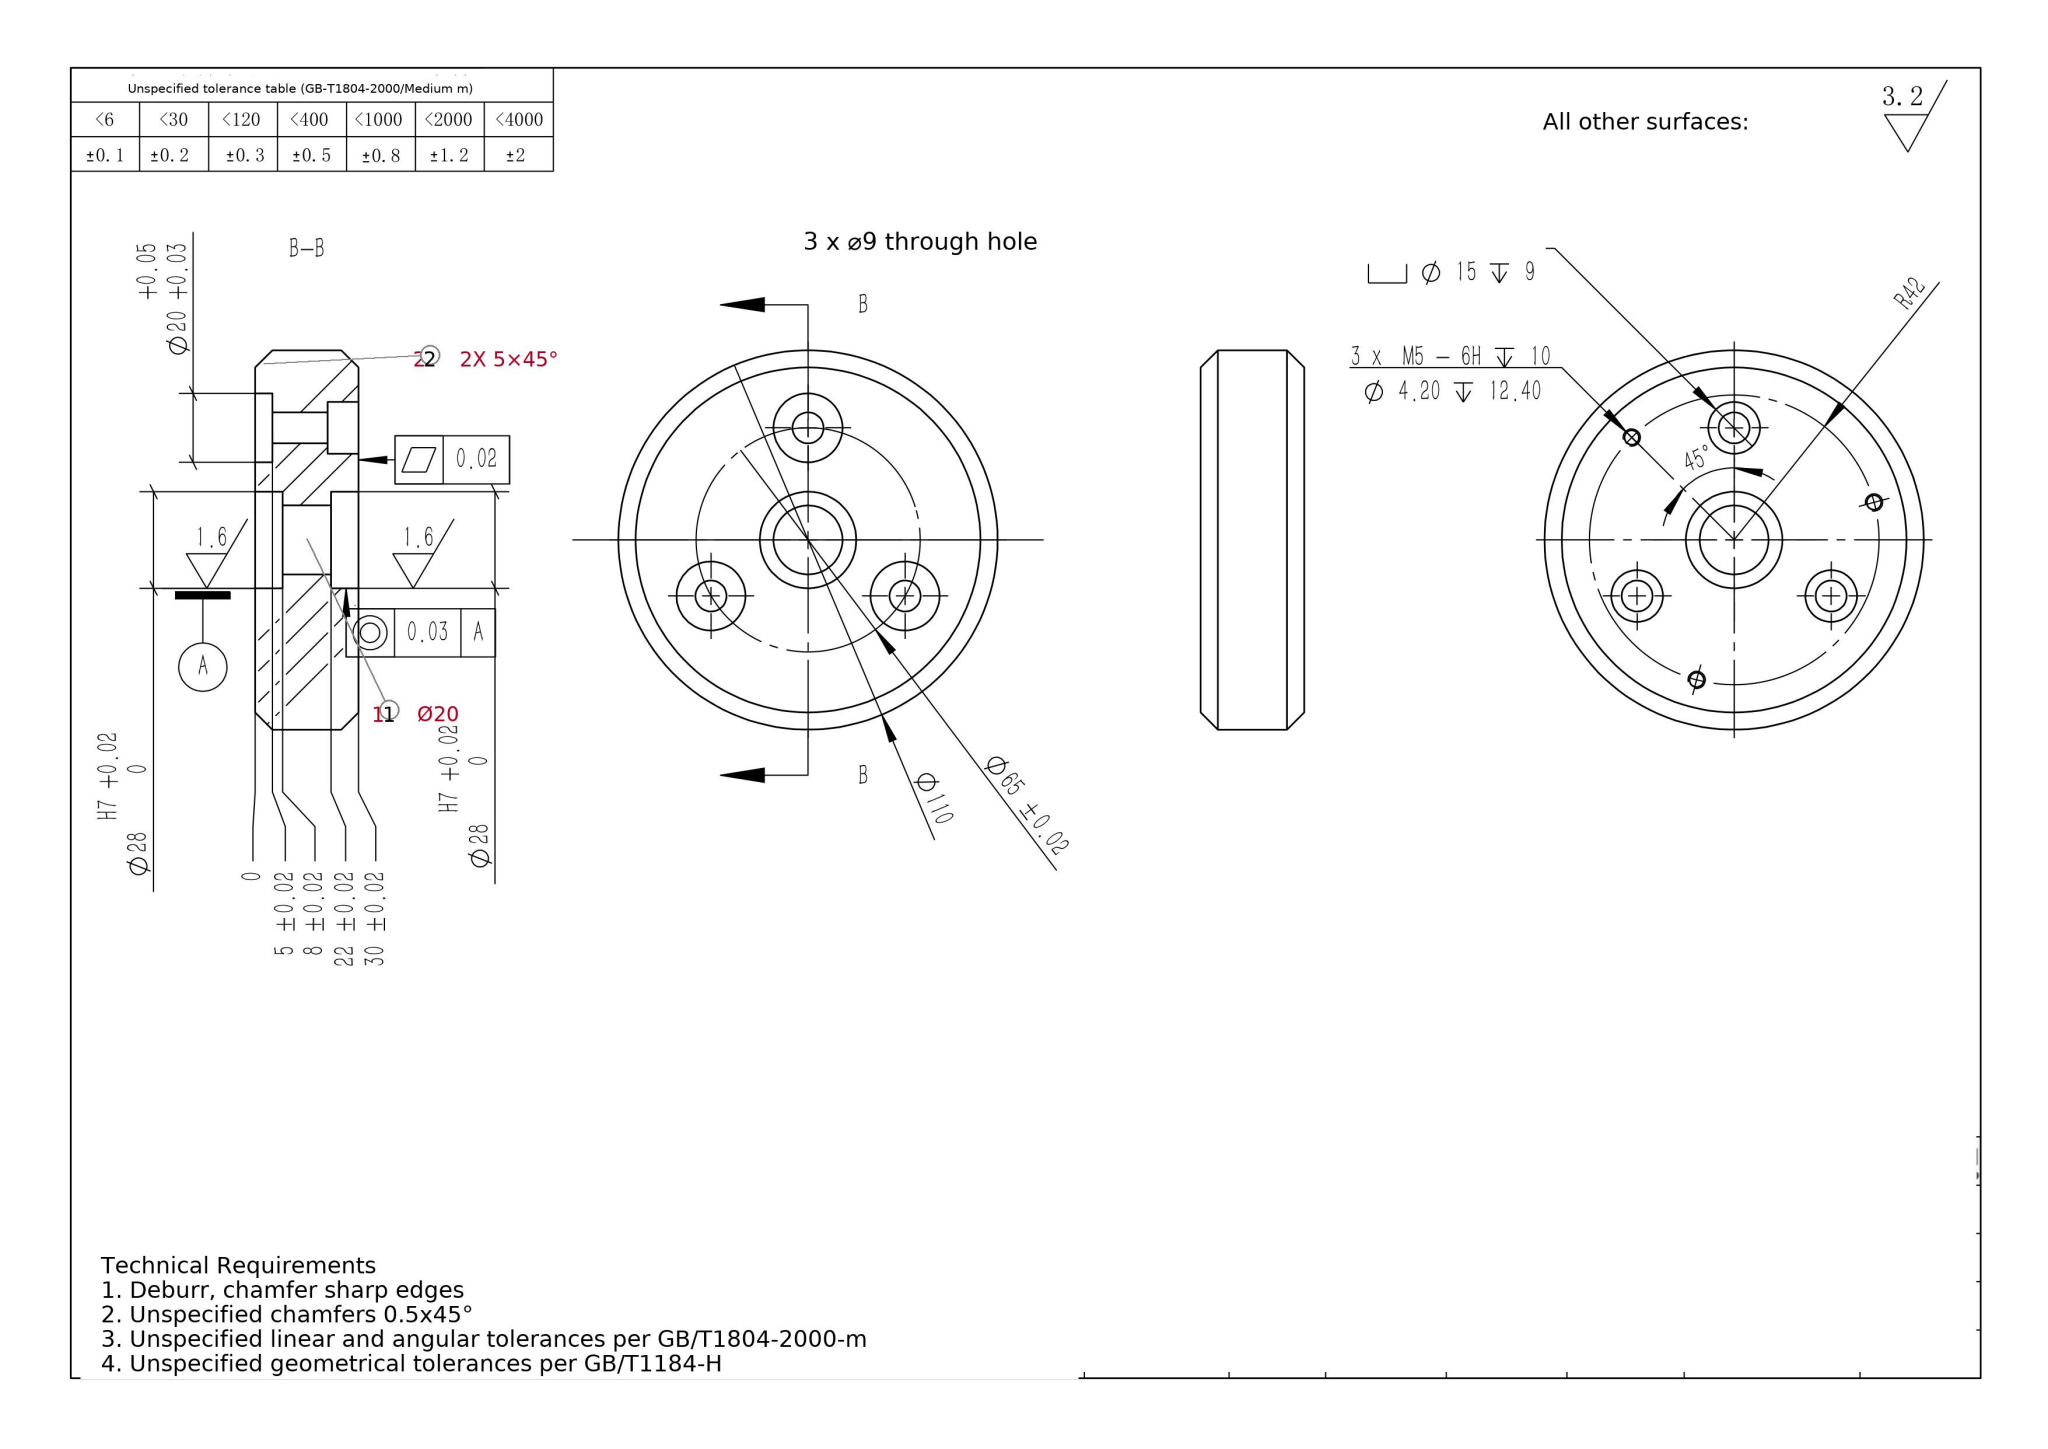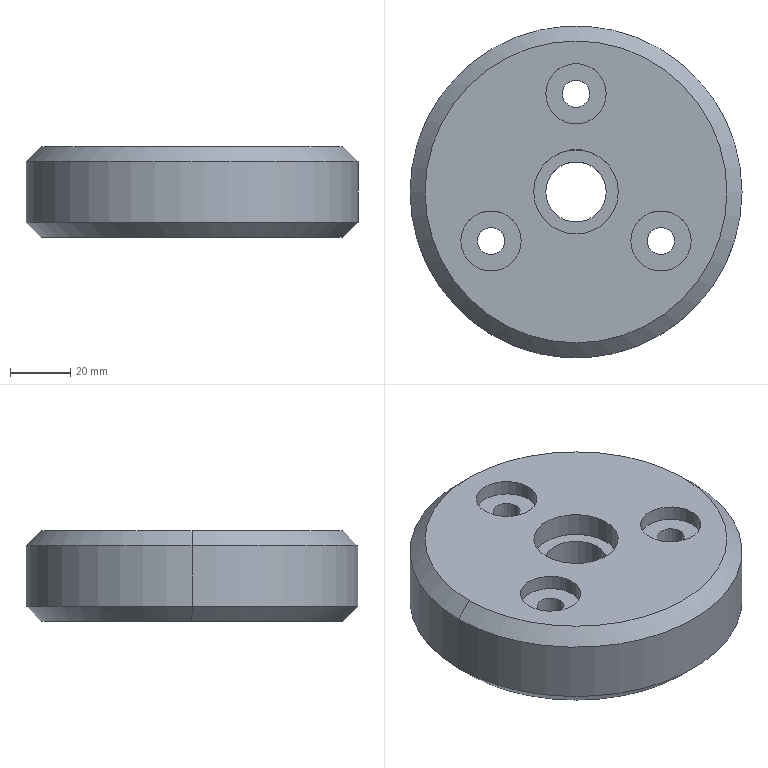Part | SolidWorks | mm | 1 solid | 52 faces | box 110 x 110 x 30 mm | volume 249402 mm3 | cylinder 32 | cone 10 | plane 10 | commonest cylinder face diameters 20 x8 4.2 x6 15 x6 9 x6 28 x4 110 x2
build123d program:
from build123d import *

# Parameters (mm, degrees)
SKETCH1_R                                         = 55
BOSS_EXTRUDE1_DEPTH                               = 30
SKETCH2_R                                         = 14
CUT_EXTRUDE1_DEPTH                                = 8
SKETCH3_R                                         = 10
CUT_EXTRUDE2_DEPTH                                = 81.833
CUT_EXTRUDE3_START                                = -8
SKETCH4_R                                         = 14
CUT_EXTRUDE3_DEPTH                                = 8
SKETCH5_R                                         = 10
CUT_EXTRUDE4_DEPTH                                = 5
HOLE_SIZE_ACCORDING_TO_HEXAGON_SOCKET_D           = 9
HOLE_SIZE_ACCORDING_TO_HEXAGON_SOCKET_CBORE_D     = 15
HOLE_SIZE_ACCORDING_TO_HEXAGON_SOCKET_CBORE_DEPTH = 9
CHAMFER1_SIZE                                     = 5
M5_TAPPED_HOLE1_D                                 = 4.2
M5_TAPPED_HOLE1_DEPTH                             = 12.4
M5_TAPPED_HOLE1_TIP                               = 1.262


with BuildPart() as part:
    # Sketch1 → Boss-Extrude1 (new body)
    with BuildSketch(Plane.XY):
        Circle(SKETCH1_R)
    extrude(amount=BOSS_EXTRUDE1_DEPTH)

    # Sketch2 → Cut-Extrude1 (cut)
    with BuildSketch(Plane.XY.offset(30)):
        Circle(SKETCH2_R)
    extrude(amount=-CUT_EXTRUDE1_DEPTH, mode=Mode.SUBTRACT)

    # Sketch3 → Cut-Extrude2 (cut, through all)
    with BuildSketch(Plane.XY.offset(22)):
        Circle(SKETCH3_R)
    extrude(amount=-CUT_EXTRUDE2_DEPTH, mode=Mode.SUBTRACT)

    # Sketch4 → Cut-Extrude3 (cut)
    with BuildSketch(Plane(origin=(0, 0, 0), x_dir=(-1, 0, 0), z_dir=(0, 0, -1)).offset(CUT_EXTRUDE3_START)):
        with Locations(Location((0, 0, 0), (0, 0, 180))):
            Circle(SKETCH4_R)
    extrude(amount=CUT_EXTRUDE3_DEPTH, mode=Mode.SUBTRACT)

    # Sketch5 → Cut-Extrude4 (cut)
    with BuildSketch(Plane.XY.offset(30)):
        with Locations((0, 32.5)):
            Circle(SKETCH5_R)
        with Locations((28.146, -16.25)):
            Circle(SKETCH5_R)
        with Locations((-28.146, -16.25)):
            Circle(SKETCH5_R)
    extrude(amount=-CUT_EXTRUDE4_DEPTH, mode=Mode.SUBTRACT)

    # Hole Size _according to_ Hexagon Socket (through all)
    with Locations(Plane(origin=(0, 0, 0), x_dir=(1, 0, 0), z_dir=(0, 0, -1))):
        with Locations((0, -32.5), (-28.146, 16.25), (28.146, 16.25)):
            CounterBoreHole(HOLE_SIZE_ACCORDING_TO_HEXAGON_SOCKET_D / 2, HOLE_SIZE_ACCORDING_TO_HEXAGON_SOCKET_CBORE_D / 2, HOLE_SIZE_ACCORDING_TO_HEXAGON_SOCKET_CBORE_DEPTH)

    # Chamfer1
    chamfer1_edges = [part.edges().sort_by_distance(p)[0] for p in [
        (-55, 0, 0),
        (-55, 0, 30),
    ]]
    chamfer(chamfer1_edges, length=CHAMFER1_SIZE)

    # M5 Tapped Hole1
    with Locations(Plane(origin=(0, 0, 0), x_dir=(-1, 0, 0), z_dir=(0, 0, -1))):
        with Locations((-29.698, 29.698), (40.569, 10.87), (-10.87, -40.569)):
            Hole(M5_TAPPED_HOLE1_D / 2, depth=M5_TAPPED_HOLE1_DEPTH)
            with Locations((0, 0, -(M5_TAPPED_HOLE1_DEPTH + M5_TAPPED_HOLE1_TIP / 2))):  # 118° drill point
                Cone(0, M5_TAPPED_HOLE1_D / 2, M5_TAPPED_HOLE1_TIP, mode=Mode.SUBTRACT)


solid = part.part